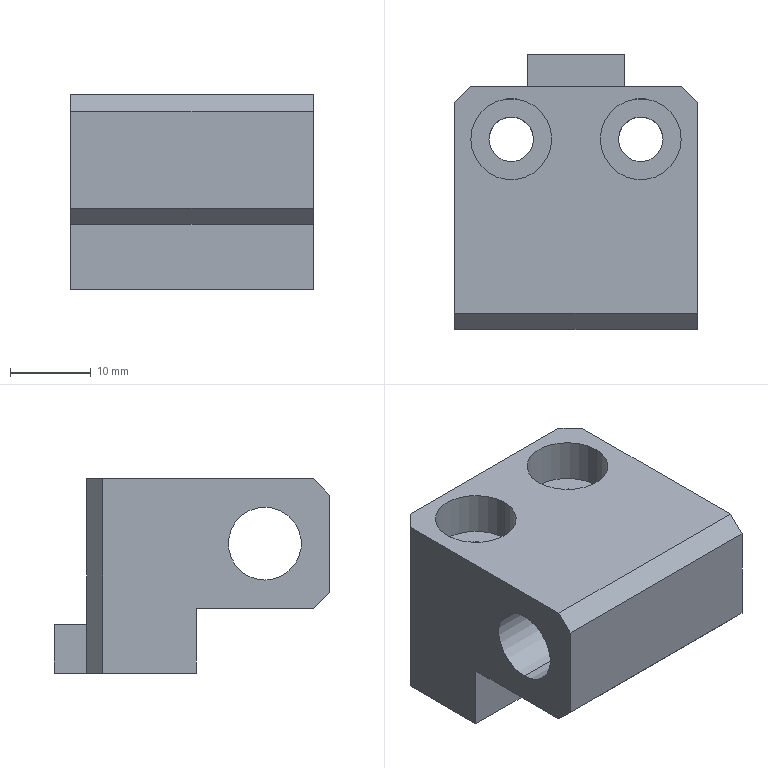Component | SolidWorks | 006GuideSeat-3 | 1 solid | 28 faces | box 30 x 34 x 24 mm | volume 14071 mm3 | plane 18 | cylinder 10 | commonest cylinder face diameters 10 x4 5.5 x4 9 x2
build123d program:
from build123d import *

# Parameters (mm, degrees)
SKETCH1_W                                            = 30
SKETCH1_H                                            = 30
BOSS_EXTRUDE1_DEPTH                                  = 24
SKETCH3_W                                            = 8
SKETCH3_H                                            = 16.5
CUT_EXTRUDE2_DEPTH                                   = 49.744
M5_HEX_SOCKET_HEAD_CAP_SCREW_COUNTERBORE_D           = 5.5
M5_HEX_SOCKET_HEAD_CAP_SCREW_COUNTERBORE_CBORE_D     = 10
M5_HEX_SOCKET_HEAD_CAP_SCREW_COUNTERBORE_CBORE_DEPTH = 5.4
SKETCH6_R                                            = 4.5
CUT_EXTRUDE3_DEPTH                                   = 49.744
CHAMFER1_SIZE                                        = 2
CHAMFER2_SIZE                                        = 2
SKETCH7_W                                            = 12
SKETCH7_H                                            = 6
BOSS_EXTRUDE2_DEPTH                                  = 4


with BuildPart() as part:
    # Sketch1 → Boss-Extrude1 (new body)
    with BuildSketch(Plane.XY):
        with Locations((15, 15)):
            Rectangle(SKETCH1_W, SKETCH1_H)
    extrude(amount=BOSS_EXTRUDE1_DEPTH)

    # Sketch3 → Cut-Extrude2 (cut, through all)
    with BuildSketch(Plane(origin=(30, 0, 0), x_dir=(0, 0, -1), z_dir=(1, 0, 0))):
        with Locations((-4, 8.25)):
            Rectangle(SKETCH3_W, SKETCH3_H)
    extrude(amount=-CUT_EXTRUDE2_DEPTH, mode=Mode.SUBTRACT)

    # M5 Hex Socket Head Cap Screw Counterbore (through all)
    with Locations(Plane.XY.offset(24)):
        with Locations((23, 23.5), (7, 23.5)):
            CounterBoreHole(M5_HEX_SOCKET_HEAD_CAP_SCREW_COUNTERBORE_D / 2, M5_HEX_SOCKET_HEAD_CAP_SCREW_COUNTERBORE_CBORE_D / 2, M5_HEX_SOCKET_HEAD_CAP_SCREW_COUNTERBORE_CBORE_DEPTH)

    # Sketch6 → Cut-Extrude3 (cut, through all)
    with BuildSketch(Plane(origin=(30, 0, 0), x_dir=(0, 0, -1), z_dir=(1, 0, 0))):
        with Locations((-16, 8)):
            Circle(SKETCH6_R)
    extrude(amount=-CUT_EXTRUDE3_DEPTH, mode=Mode.SUBTRACT)

    # Chamfer1
    chamfer1_edges = [part.edges().sort_by_distance(p)[0] for p in [
        (15, 0, 8),
        (15, 0, 24),
    ]]
    chamfer(chamfer1_edges, length=CHAMFER1_SIZE)

    # Chamfer2
    chamfer2_edges = [part.edges().sort_by_distance(p)[0] for p in [
        (0, 30, 12),
        (30, 30, 12),
    ]]
    chamfer(chamfer2_edges, length=CHAMFER2_SIZE)

    # Sketch7 → Boss-Extrude2 (add)
    with BuildSketch(Plane(origin=(0, 30, 0), x_dir=(1, 0, 0), z_dir=(0, 1, 0))):
        with Locations((15, -3)):
            Rectangle(SKETCH7_W, SKETCH7_H)
    extrude(amount=BOSS_EXTRUDE2_DEPTH)


solid = part.part

# Placed as in the assembly
solid = solid.moved(Location((-135.796, 16.924, 37.04), (0, 0, 0)))
STEP:
#1=CARTESIAN_POINT('',(-5.346,0.9813,2.265));
#2=VERTEX_POINT('',#1);
#3=CARTESIAN_POINT('',(-5.346,0.9813,1.911));
#4=VERTEX_POINT('',#3);
#5=CARTESIAN_POINT('',(-5.346,0.9813,2.088));
#6=DIRECTION('',(1.,0.,0.));
#7=DIRECTION('',(0.,0.,-1.));
#8=AXIS2_PLACEMENT_3D('',#5,#6,#7);
#9=CIRCLE('',#8,0.1772);
#10=EDGE_CURVE('',#2,#4,#9,.T.);
#11=ORIENTED_EDGE('',*,*,#10,.F.);
#12=CARTESIAN_POINT('',(-4.165,0.9813,2.265));
#13=VERTEX_POINT('',#12);
#14=CARTESIAN_POINT('',(-5.346,0.9813,2.265));
#15=DIRECTION('',(1.,0.,0.));
#16=VECTOR('',#15,39.37);
#17=LINE('',#14,#16);
#18=EDGE_CURVE('',#2,#13,#17,.T.);
#19=ORIENTED_EDGE('',*,*,#18,.T.);
#20=CARTESIAN_POINT('',(-4.165,0.9813,1.911));
#21=VERTEX_POINT('',#20);
#22=CARTESIAN_POINT('',(-4.165,0.9813,2.088));
#23=DIRECTION('',(1.,0.,0.));
#24=DIRECTION('',(0.,0.,-1.));
#25=AXIS2_PLACEMENT_3D('',#22,#23,#24);
#26=CIRCLE('',#25,0.1772);
#27=EDGE_CURVE('',#13,#21,#26,.T.);
#28=ORIENTED_EDGE('',*,*,#27,.T.);
#29=CARTESIAN_POINT('',(-5.346,0.9813,1.911));
#30=DIRECTION('',(1.,0.,0.));
#31=VECTOR('',#30,39.37);
#32=LINE('',#29,#31);
#33=EDGE_CURVE('',#4,#21,#32,.T.);
#34=ORIENTED_EDGE('',*,*,#33,.F.);
#35=EDGE_LOOP('',(#11,#19,#28,#34));
#36=FACE_OUTER_BOUND('',#35,.T.);
#37=CARTESIAN_POINT('',(-5.346,0.9813,2.088));
#38=DIRECTION('',(1.,0.,0.));
#39=DIRECTION('',(0.,0.,-1.));
#40=AXIS2_PLACEMENT_3D('',#37,#38,#39);
#41=CYLINDRICAL_SURFACE('',#40,0.1772);
#42=ADVANCED_FACE('',(#36),#41,.F.);
#43=CARTESIAN_POINT('',(-4.638,1.592,2.191));
#44=VERTEX_POINT('',#43);
#45=CARTESIAN_POINT('',(-4.244,1.592,2.191));
#46=VERTEX_POINT('',#45);
#47=CARTESIAN_POINT('',(-4.441,1.592,2.191));
#48=DIRECTION('',(0.,0.,1.));
#49=DIRECTION('',(1.,0.,0.));
#50=AXIS2_PLACEMENT_3D('',#47,#48,#49);
#51=CIRCLE('',#50,0.1969);
#52=EDGE_CURVE('',#44,#46,#51,.T.);
#53=ORIENTED_EDGE('',*,*,#52,.F.);
#54=CARTESIAN_POINT('',(-4.638,1.592,2.403));
#55=VERTEX_POINT('',#54);
#56=CARTESIAN_POINT('',(-4.638,1.592,2.403));
#57=DIRECTION('',(0.,0.,1.));
#58=VECTOR('',#57,39.37);
#59=LINE('',#56,#58);
#60=EDGE_CURVE('',#44,#55,#59,.T.);
#61=ORIENTED_EDGE('',*,*,#60,.T.);
#62=CARTESIAN_POINT('',(-4.244,1.592,2.403));
#63=VERTEX_POINT('',#62);
#64=CARTESIAN_POINT('',(-4.441,1.592,2.403));
#65=DIRECTION('',(0.,0.,1.));
#66=DIRECTION('',(1.,0.,0.));
#67=AXIS2_PLACEMENT_3D('',#64,#65,#66);
#68=CIRCLE('',#67,0.1969);
#69=EDGE_CURVE('',#55,#63,#68,.T.);
#70=ORIENTED_EDGE('',*,*,#69,.T.);
#71=CARTESIAN_POINT('',(-4.244,1.592,2.403));
#72=DIRECTION('',(0.,0.,1.));
#73=VECTOR('',#72,39.37);
#74=LINE('',#71,#73);
#75=EDGE_CURVE('',#46,#63,#74,.T.);
#76=ORIENTED_EDGE('',*,*,#75,.F.);
#77=EDGE_LOOP('',(#53,#61,#70,#76));
#78=FACE_OUTER_BOUND('',#77,.T.);
#79=CARTESIAN_POINT('',(-4.441,1.592,2.403));
#80=DIRECTION('',(0.,0.,1.));
#81=DIRECTION('',(1.,0.,0.));
#82=AXIS2_PLACEMENT_3D('',#79,#80,#81);
#83=CYLINDRICAL_SURFACE('',#82,0.1969);
#84=ADVANCED_FACE('',(#78),#83,.F.);
#85=CARTESIAN_POINT('',(-4.549,1.592,1.458));
#86=VERTEX_POINT('',#85);
#87=CARTESIAN_POINT('',(-4.333,1.592,1.458));
#88=VERTEX_POINT('',#87);
#89=CARTESIAN_POINT('',(-4.441,1.592,1.458));
#90=DIRECTION('',(0.,0.,1.));
#91=DIRECTION('',(1.,0.,0.));
#92=AXIS2_PLACEMENT_3D('',#89,#90,#91);
#93=CIRCLE('',#92,0.1083);
#94=EDGE_CURVE('',#86,#88,#93,.T.);
#95=ORIENTED_EDGE('',*,*,#94,.F.);
#96=CARTESIAN_POINT('',(-4.549,1.592,2.191));
#97=VERTEX_POINT('',#96);
#98=CARTESIAN_POINT('',(-4.549,1.592,2.403));
#99=DIRECTION('',(0.,0.,1.));
#100=VECTOR('',#99,39.37);
#101=LINE('',#98,#100);
#102=EDGE_CURVE('',#86,#97,#101,.T.);
#103=ORIENTED_EDGE('',*,*,#102,.T.);
#104=CARTESIAN_POINT('',(-4.333,1.592,2.191));
#105=VERTEX_POINT('',#104);
#106=CARTESIAN_POINT('',(-4.441,1.592,2.191));
#107=DIRECTION('',(0.,0.,1.));
#108=DIRECTION('',(1.,0.,0.));
#109=AXIS2_PLACEMENT_3D('',#106,#107,#108);
#110=CIRCLE('',#109,0.1083);
#111=EDGE_CURVE('',#97,#105,#110,.T.);
#112=ORIENTED_EDGE('',*,*,#111,.T.);
#113=CARTESIAN_POINT('',(-4.333,1.592,2.403));
#114=DIRECTION('',(0.,0.,1.));
#115=VECTOR('',#114,39.37);
#116=LINE('',#113,#115);
#117=EDGE_CURVE('',#88,#105,#116,.T.);
#118=ORIENTED_EDGE('',*,*,#117,.F.);
#119=EDGE_LOOP('',(#95,#103,#112,#118));
#120=FACE_OUTER_BOUND('',#119,.T.);
#121=CARTESIAN_POINT('',(-4.441,1.592,2.403));
#122=DIRECTION('',(0.,0.,1.));
#123=DIRECTION('',(1.,0.,0.));
#124=AXIS2_PLACEMENT_3D('',#121,#122,#123);
#125=CYLINDRICAL_SURFACE('',#124,0.1083);
#126=ADVANCED_FACE('',(#120),#125,.F.);
#127=CARTESIAN_POINT('',(-5.268,1.592,2.191));
#128=VERTEX_POINT('',#127);
#129=CARTESIAN_POINT('',(-4.874,1.592,2.191));
#130=VERTEX_POINT('',#129);
#131=CARTESIAN_POINT('',(-5.071,1.592,2.191));
#132=DIRECTION('',(0.,0.,1.));
#133=DIRECTION('',(1.,0.,0.));
#134=AXIS2_PLACEMENT_3D('',#131,#132,#133);
#135=CIRCLE('',#134,0.1969);
#136=EDGE_CURVE('',#128,#130,#135,.T.);
#137=ORIENTED_EDGE('',*,*,#136,.F.);
#138=CARTESIAN_POINT('',(-5.268,1.592,2.403));
#139=VERTEX_POINT('',#138);
#140=CARTESIAN_POINT('',(-5.268,1.592,2.403));
#141=DIRECTION('',(0.,0.,1.));
#142=VECTOR('',#141,39.37);
#143=LINE('',#140,#142);
#144=EDGE_CURVE('',#128,#139,#143,.T.);
#145=ORIENTED_EDGE('',*,*,#144,.T.);
#146=CARTESIAN_POINT('',(-4.874,1.592,2.403));
#147=VERTEX_POINT('',#146);
#148=CARTESIAN_POINT('',(-5.071,1.592,2.403));
#149=DIRECTION('',(0.,0.,1.));
#150=DIRECTION('',(1.,0.,0.));
#151=AXIS2_PLACEMENT_3D('',#148,#149,#150);
#152=CIRCLE('',#151,0.1969);
#153=EDGE_CURVE('',#139,#147,#152,.T.);
#154=ORIENTED_EDGE('',*,*,#153,.T.);
#155=CARTESIAN_POINT('',(-4.874,1.592,2.403));
#156=DIRECTION('',(0.,0.,1.));
#157=VECTOR('',#156,39.37);
#158=LINE('',#155,#157);
#159=EDGE_CURVE('',#130,#147,#158,.T.);
#160=ORIENTED_EDGE('',*,*,#159,.F.);
#161=EDGE_LOOP('',(#137,#145,#154,#160));
#162=FACE_OUTER_BOUND('',#161,.T.);
#163=CARTESIAN_POINT('',(-5.071,1.592,2.403));
#164=DIRECTION('',(0.,0.,1.));
#165=DIRECTION('',(1.,0.,0.));
#166=AXIS2_PLACEMENT_3D('',#163,#164,#165);
#167=CYLINDRICAL_SURFACE('',#166,0.1969);
#168=ADVANCED_FACE('',(#162),#167,.F.);
#169=CARTESIAN_POINT('',(-5.179,1.592,1.458));
#170=VERTEX_POINT('',#169);
#171=CARTESIAN_POINT('',(-4.962,1.592,1.458));
#172=VERTEX_POINT('',#171);
#173=CARTESIAN_POINT('',(-5.071,1.592,1.458));
#174=DIRECTION('',(0.,0.,1.));
#175=DIRECTION('',(1.,0.,0.));
#176=AXIS2_PLACEMENT_3D('',#173,#174,#175);
#177=CIRCLE('',#176,0.1083);
#178=EDGE_CURVE('',#170,#172,#177,.T.);
#179=ORIENTED_EDGE('',*,*,#178,.F.);
#180=CARTESIAN_POINT('',(-5.179,1.592,2.191));
#181=VERTEX_POINT('',#180);
#182=CARTESIAN_POINT('',(-5.179,1.592,2.403));
#183=DIRECTION('',(0.,0.,1.));
#184=VECTOR('',#183,39.37);
#185=LINE('',#182,#184);
#186=EDGE_CURVE('',#170,#181,#185,.T.);
#187=ORIENTED_EDGE('',*,*,#186,.T.);
#188=CARTESIAN_POINT('',(-4.962,1.592,2.191));
#189=VERTEX_POINT('',#188);
#190=CARTESIAN_POINT('',(-5.071,1.592,2.191));
#191=DIRECTION('',(0.,0.,1.));
#192=DIRECTION('',(1.,0.,0.));
#193=AXIS2_PLACEMENT_3D('',#190,#191,#192);
#194=CIRCLE('',#193,0.1083);
#195=EDGE_CURVE('',#181,#189,#194,.T.);
#196=ORIENTED_EDGE('',*,*,#195,.T.);
#197=CARTESIAN_POINT('',(-4.962,1.592,2.403));
#198=DIRECTION('',(0.,0.,1.));
#199=VECTOR('',#198,39.37);
#200=LINE('',#197,#199);
#201=EDGE_CURVE('',#172,#189,#200,.T.);
#202=ORIENTED_EDGE('',*,*,#201,.F.);
#203=EDGE_LOOP('',(#179,#187,#196,#202));
#204=FACE_OUTER_BOUND('',#203,.T.);
#205=CARTESIAN_POINT('',(-5.071,1.592,2.403));
#206=DIRECTION('',(0.,0.,1.));
#207=DIRECTION('',(1.,0.,0.));
#208=AXIS2_PLACEMENT_3D('',#205,#206,#207);
#209=CYLINDRICAL_SURFACE('',#208,0.1083);
#210=ADVANCED_FACE('',(#204),#209,.F.);
#211=CARTESIAN_POINT('',(-4.992,1.847,1.458));
#212=VERTEX_POINT('',#211);
#213=CARTESIAN_POINT('',(-4.992,1.847,1.695));
#214=VERTEX_POINT('',#213);
#215=CARTESIAN_POINT('',(-4.992,1.847,1.458));
#216=DIRECTION('',(0.,0.,1.));
#217=VECTOR('',#216,39.37);
#218=LINE('',#215,#217);
#219=EDGE_CURVE('',#212,#214,#218,.T.);
#220=ORIENTED_EDGE('',*,*,#219,.F.);
#221=CARTESIAN_POINT('',(-5.268,1.847,1.458));
#222=VERTEX_POINT('',#221);
#223=CARTESIAN_POINT('',(-5.346,1.847,1.458));
#224=DIRECTION('',(-1.,0.,0.));
#225=VECTOR('',#224,39.37);
#226=LINE('',#223,#225);
#227=EDGE_CURVE('',#212,#222,#226,.T.);
#228=ORIENTED_EDGE('',*,*,#227,.T.);
#229=CARTESIAN_POINT('',(-5.268,1.847,2.403));
#230=VERTEX_POINT('',#229);
#231=CARTESIAN_POINT('',(-5.268,1.847,2.403));
#232=DIRECTION('',(0.,0.,1.));
#233=VECTOR('',#232,39.37);
#234=LINE('',#231,#233);
#235=EDGE_CURVE('',#222,#230,#234,.T.);
#236=ORIENTED_EDGE('',*,*,#235,.T.);
#237=CARTESIAN_POINT('',(-4.244,1.847,2.403));
#238=VERTEX_POINT('',#237);
#239=CARTESIAN_POINT('',(-5.346,1.847,2.403));
#240=DIRECTION('',(-1.,0.,0.));
#241=VECTOR('',#240,39.37);
#242=LINE('',#239,#241);
#243=EDGE_CURVE('',#238,#230,#242,.T.);
#244=ORIENTED_EDGE('',*,*,#243,.F.);
#245=CARTESIAN_POINT('',(-4.244,1.847,1.458));
#246=VERTEX_POINT('',#245);
#247=CARTESIAN_POINT('',(-4.244,1.847,2.403));
#248=DIRECTION('',(0.,0.,-1.));
#249=VECTOR('',#248,39.37);
#250=LINE('',#247,#249);
#251=EDGE_CURVE('',#238,#246,#250,.T.);
#252=ORIENTED_EDGE('',*,*,#251,.T.);
#253=CARTESIAN_POINT('',(-4.52,1.847,1.458));
#254=VERTEX_POINT('',#253);
#255=CARTESIAN_POINT('',(-5.346,1.847,1.458));
#256=DIRECTION('',(-1.,0.,0.));
#257=VECTOR('',#256,39.37);
#258=LINE('',#255,#257);
#259=EDGE_CURVE('',#246,#254,#258,.T.);
#260=ORIENTED_EDGE('',*,*,#259,.T.);
#261=CARTESIAN_POINT('',(-4.52,1.847,1.695));
#262=VERTEX_POINT('',#261);
#263=CARTESIAN_POINT('',(-4.52,1.847,1.458));
#264=DIRECTION('',(0.,0.,-1.));
#265=VECTOR('',#264,39.37);
#266=LINE('',#263,#265);
#267=EDGE_CURVE('',#262,#254,#266,.T.);
#268=ORIENTED_EDGE('',*,*,#267,.F.);
#269=CARTESIAN_POINT('',(-4.992,1.847,1.695));
#270=DIRECTION('',(1.,0.,0.));
#271=VECTOR('',#270,39.37);
#272=LINE('',#269,#271);
#273=EDGE_CURVE('',#214,#262,#272,.T.);
#274=ORIENTED_EDGE('',*,*,#273,.F.);
#275=EDGE_LOOP('',(#220,#228,#236,#244,#252,#260,#268,#274));
#276=FACE_OUTER_BOUND('',#275,.T.);
#277=CARTESIAN_POINT('',(-5.346,1.847,2.403));
#278=DIRECTION('',(0.,-1.,0.));
#279=DIRECTION('',(0.,0.,-1.));
#280=AXIS2_PLACEMENT_3D('',#277,#278,#279);
#281=PLANE('',#280);
#282=ADVANCED_FACE('',(#276),#281,.F.);
#283=CARTESIAN_POINT('',(-5.346,0.9813,2.088));
#284=DIRECTION('',(1.,0.,0.));
#285=DIRECTION('',(0.,0.,-1.));
#286=AXIS2_PLACEMENT_3D('',#283,#284,#285);
#287=CIRCLE('',#286,0.1772);
#288=EDGE_CURVE('',#4,#2,#287,.T.);
#289=ORIENTED_EDGE('',*,*,#288,.T.);
#290=ORIENTED_EDGE('',*,*,#10,.T.);
#291=EDGE_LOOP('',(#289,#290));
#292=FACE_BOUND('',#291,.T.);
#293=CARTESIAN_POINT('',(-5.346,1.769,2.403));
#294=VERTEX_POINT('',#293);
#295=CARTESIAN_POINT('',(-5.346,0.7451,2.403));
#296=VERTEX_POINT('',#295);
#297=CARTESIAN_POINT('',(-5.346,0.6663,2.403));
#298=DIRECTION('',(0.,-1.,0.));
#299=VECTOR('',#298,39.37);
#300=LINE('',#297,#299);
#301=EDGE_CURVE('',#294,#296,#300,.T.);
#302=ORIENTED_EDGE('',*,*,#301,.F.);
#303=CARTESIAN_POINT('',(-5.346,1.769,1.458));
#304=VERTEX_POINT('',#303);
#305=CARTESIAN_POINT('',(-5.346,1.769,2.403));
#306=DIRECTION('',(0.,0.,-1.));
#307=VECTOR('',#306,39.37);
#308=LINE('',#305,#307);
#309=EDGE_CURVE('',#294,#304,#308,.T.);
#310=ORIENTED_EDGE('',*,*,#309,.T.);
#311=CARTESIAN_POINT('',(-5.346,1.316,1.458));
#312=VERTEX_POINT('',#311);
#313=CARTESIAN_POINT('',(-5.346,0.6663,1.458));
#314=DIRECTION('',(0.,-1.,0.));
#315=VECTOR('',#314,39.37);
#316=LINE('',#313,#315);
#317=EDGE_CURVE('',#304,#312,#316,.T.);
#318=ORIENTED_EDGE('',*,*,#317,.T.);
#319=CARTESIAN_POINT('',(-5.346,1.316,1.773));
#320=VERTEX_POINT('',#319);
#321=CARTESIAN_POINT('',(-5.346,1.316,1.458));
#322=DIRECTION('',(0.,0.,1.));
#323=VECTOR('',#322,39.37);
#324=LINE('',#321,#323);
#325=EDGE_CURVE('',#312,#320,#324,.T.);
#326=ORIENTED_EDGE('',*,*,#325,.T.);
#327=CARTESIAN_POINT('',(-5.346,0.7451,1.773));
#328=VERTEX_POINT('',#327);
#329=CARTESIAN_POINT('',(-5.346,0.6663,1.773));
#330=DIRECTION('',(0.,-1.,0.));
#331=VECTOR('',#330,39.37);
#332=LINE('',#329,#331);
#333=EDGE_CURVE('',#320,#328,#332,.T.);
#334=ORIENTED_EDGE('',*,*,#333,.T.);
#335=CARTESIAN_POINT('',(-5.346,0.6663,1.852));
#336=VERTEX_POINT('',#335);
#337=CARTESIAN_POINT('',(-5.346,0.6663,1.852));
#338=DIRECTION('',(0.,-0.7071,0.7071));
#339=VECTOR('',#338,39.37);
#340=LINE('',#337,#339);
#341=EDGE_CURVE('',#328,#336,#340,.T.);
#342=ORIENTED_EDGE('',*,*,#341,.T.);
#343=CARTESIAN_POINT('',(-5.346,0.6663,2.324));
#344=VERTEX_POINT('',#343);
#345=CARTESIAN_POINT('',(-5.346,0.6663,2.403));
#346=DIRECTION('',(0.,0.,-1.));
#347=VECTOR('',#346,39.37);
#348=LINE('',#345,#347);
#349=EDGE_CURVE('',#344,#336,#348,.T.);
#350=ORIENTED_EDGE('',*,*,#349,.F.);
#351=CARTESIAN_POINT('',(-5.346,0.7451,2.403));
#352=DIRECTION('',(0.,0.7071,0.7071));
#353=VECTOR('',#352,39.37);
#354=LINE('',#351,#353);
#355=EDGE_CURVE('',#344,#296,#354,.T.);
#356=ORIENTED_EDGE('',*,*,#355,.T.);
#357=EDGE_LOOP('',(#302,#310,#318,#326,#334,#342,#350,#356));
#358=FACE_OUTER_BOUND('',#357,.T.);
#359=CARTESIAN_POINT('',(-5.346,0.6663,2.403));
#360=DIRECTION('',(1.,0.,0.));
#361=DIRECTION('',(0.,0.,-1.));
#362=AXIS2_PLACEMENT_3D('',#359,#360,#361);
#363=PLANE('',#362);
#364=ADVANCED_FACE('',(#292,#358),#363,.F.);
#365=ORIENTED_EDGE('',*,*,#349,.T.);
#366=CARTESIAN_POINT('',(-4.165,0.6663,1.852));
#367=VERTEX_POINT('',#366);
#368=CARTESIAN_POINT('',(-5.346,0.6663,1.852));
#369=DIRECTION('',(1.,0.,0.));
#370=VECTOR('',#369,39.37);
#371=LINE('',#368,#370);
#372=EDGE_CURVE('',#336,#367,#371,.T.);
#373=ORIENTED_EDGE('',*,*,#372,.T.);
#374=CARTESIAN_POINT('',(-4.165,0.6663,2.324));
#375=VERTEX_POINT('',#374);
#376=CARTESIAN_POINT('',(-4.165,0.6663,2.403));
#377=DIRECTION('',(0.,0.,-1.));
#378=VECTOR('',#377,39.37);
#379=LINE('',#376,#378);
#380=EDGE_CURVE('',#375,#367,#379,.T.);
#381=ORIENTED_EDGE('',*,*,#380,.F.);
#382=CARTESIAN_POINT('',(-5.346,0.6663,2.324));
#383=DIRECTION('',(-1.,0.,0.));
#384=VECTOR('',#383,39.37);
#385=LINE('',#382,#384);
#386=EDGE_CURVE('',#375,#344,#385,.T.);
#387=ORIENTED_EDGE('',*,*,#386,.T.);
#388=EDGE_LOOP('',(#365,#373,#381,#387));
#389=FACE_OUTER_BOUND('',#388,.T.);
#390=CARTESIAN_POINT('',(-5.346,0.6663,2.403));
#391=DIRECTION('',(0.,1.,0.));
#392=DIRECTION('',(0.,0.,1.));
#393=AXIS2_PLACEMENT_3D('',#390,#391,#392);
#394=PLANE('',#393);
#395=ADVANCED_FACE('',(#389),#394,.F.);
#396=CARTESIAN_POINT('',(-4.165,0.9813,2.088));
#397=DIRECTION('',(1.,0.,0.));
#398=DIRECTION('',(0.,0.,-1.));
#399=AXIS2_PLACEMENT_3D('',#396,#397,#398);
#400=CIRCLE('',#399,0.1772);
#401=EDGE_CURVE('',#21,#13,#400,.T.);
#402=ORIENTED_EDGE('',*,*,#401,.F.);
#403=ORIENTED_EDGE('',*,*,#27,.F.);
#404=EDGE_LOOP('',(#402,#403));
#405=FACE_BOUND('',#404,.T.);
#406=CARTESIAN_POINT('',(-4.165,1.316,1.458));
#407=VERTEX_POINT('',#406);
#408=CARTESIAN_POINT('',(-4.165,1.769,1.458));
#409=VERTEX_POINT('',#408);
#410=CARTESIAN_POINT('',(-4.165,0.6663,1.458));
#411=DIRECTION('',(0.,1.,0.));
#412=VECTOR('',#411,39.37);
#413=LINE('',#410,#412);
#414=EDGE_CURVE('',#407,#409,#413,.T.);
#415=ORIENTED_EDGE('',*,*,#414,.T.);
#416=CARTESIAN_POINT('',(-4.165,1.769,2.403));
#417=VERTEX_POINT('',#416);
#418=CARTESIAN_POINT('',(-4.165,1.769,2.403));
#419=DIRECTION('',(0.,0.,1.));
#420=VECTOR('',#419,39.37);
#421=LINE('',#418,#420);
#422=EDGE_CURVE('',#409,#417,#421,.T.);
#423=ORIENTED_EDGE('',*,*,#422,.T.);
#424=CARTESIAN_POINT('',(-4.165,0.7451,2.403));
#425=VERTEX_POINT('',#424);
#426=CARTESIAN_POINT('',(-4.165,0.6663,2.403));
#427=DIRECTION('',(0.,1.,0.));
#428=VECTOR('',#427,39.37);
#429=LINE('',#426,#428);
#430=EDGE_CURVE('',#425,#417,#429,.T.);
#431=ORIENTED_EDGE('',*,*,#430,.F.);
#432=CARTESIAN_POINT('',(-4.165,0.7451,2.403));
#433=DIRECTION('',(0.,-0.7071,-0.7071));
#434=VECTOR('',#433,39.37);
#435=LINE('',#432,#434);
#436=EDGE_CURVE('',#425,#375,#435,.T.);
#437=ORIENTED_EDGE('',*,*,#436,.T.);
#438=ORIENTED_EDGE('',*,*,#380,.T.);
#439=CARTESIAN_POINT('',(-4.165,0.7451,1.773));
#440=VERTEX_POINT('',#439);
#441=CARTESIAN_POINT('',(-4.165,0.6663,1.852));
#442=DIRECTION('',(0.,0.7071,-0.7071));
#443=VECTOR('',#442,39.37);
#444=LINE('',#441,#443);
#445=EDGE_CURVE('',#367,#440,#444,.T.);
#446=ORIENTED_EDGE('',*,*,#445,.T.);
#447=CARTESIAN_POINT('',(-4.165,1.316,1.773));
#448=VERTEX_POINT('',#447);
#449=CARTESIAN_POINT('',(-4.165,0.6663,1.773));
#450=DIRECTION('',(0.,-1.,0.));
#451=VECTOR('',#450,39.37);
#452=LINE('',#449,#451);
#453=EDGE_CURVE('',#448,#440,#452,.T.);
#454=ORIENTED_EDGE('',*,*,#453,.F.);
#455=CARTESIAN_POINT('',(-4.165,1.316,1.458));
#456=DIRECTION('',(0.,0.,1.));
#457=VECTOR('',#456,39.37);
#458=LINE('',#455,#457);
#459=EDGE_CURVE('',#407,#448,#458,.T.);
#460=ORIENTED_EDGE('',*,*,#459,.F.);
#461=EDGE_LOOP('',(#415,#423,#431,#437,#438,#446,#454,#460));
#462=FACE_OUTER_BOUND('',#461,.T.);
#463=CARTESIAN_POINT('',(-4.165,0.6663,2.403));
#464=DIRECTION('',(-1.,0.,0.));
#465=DIRECTION('',(0.,0.,1.));
#466=AXIS2_PLACEMENT_3D('',#463,#464,#465);
#467=PLANE('',#466);
#468=ADVANCED_FACE('',(#405,#462),#467,.F.);
#469=CARTESIAN_POINT('',(-4.441,1.592,2.403));
#470=DIRECTION('',(0.,0.,1.));
#471=DIRECTION('',(1.,0.,0.));
#472=AXIS2_PLACEMENT_3D('',#469,#470,#471);
#473=CIRCLE('',#472,0.1969);
#474=EDGE_CURVE('',#63,#55,#473,.T.);
#475=ORIENTED_EDGE('',*,*,#474,.F.);
#476=ORIENTED_EDGE('',*,*,#69,.F.);
#477=EDGE_LOOP('',(#475,#476));
#478=FACE_BOUND('',#477,.T.);
#479=CARTESIAN_POINT('',(-5.071,1.592,2.403));
#480=DIRECTION('',(0.,0.,1.));
#481=DIRECTION('',(1.,0.,0.));
#482=AXIS2_PLACEMENT_3D('',#479,#480,#481);
#483=CIRCLE('',#482,0.1969);
#484=EDGE_CURVE('',#147,#139,#483,.T.);
#485=ORIENTED_EDGE('',*,*,#484,.F.);
#486=ORIENTED_EDGE('',*,*,#153,.F.);
#487=EDGE_LOOP('',(#485,#486));
#488=FACE_BOUND('',#487,.T.);
#489=ORIENTED_EDGE('',*,*,#243,.T.);
#490=CARTESIAN_POINT('',(-5.346,1.769,2.403));
#491=DIRECTION('',(-0.7071,-0.7071,0.));
#492=VECTOR('',#491,39.37);
#493=LINE('',#490,#492);
#494=EDGE_CURVE('',#230,#294,#493,.T.);
#495=ORIENTED_EDGE('',*,*,#494,.T.);
#496=ORIENTED_EDGE('',*,*,#301,.T.);
#497=CARTESIAN_POINT('',(-5.346,0.7451,2.403));
#498=DIRECTION('',(1.,0.,0.));
#499=VECTOR('',#498,39.37);
#500=LINE('',#497,#499);
#501=EDGE_CURVE('',#296,#425,#500,.T.);
#502=ORIENTED_EDGE('',*,*,#501,.T.);
#503=ORIENTED_EDGE('',*,*,#430,.T.);
#504=CARTESIAN_POINT('',(-4.244,1.847,2.403));
#505=DIRECTION('',(-0.7071,0.7071,0.));
#506=VECTOR('',#505,39.37);
#507=LINE('',#504,#506);
#508=EDGE_CURVE('',#417,#238,#507,.T.);
#509=ORIENTED_EDGE('',*,*,#508,.T.);
#510=EDGE_LOOP('',(#489,#495,#496,#502,#503,#509));
#511=FACE_OUTER_BOUND('',#510,.T.);
#512=CARTESIAN_POINT('',(-5.346,0.6663,2.403));
#513=DIRECTION('',(0.,0.,-1.));
#514=DIRECTION('',(-1.,0.,0.));
#515=AXIS2_PLACEMENT_3D('',#512,#513,#514);
#516=PLANE('',#515);
#517=ADVANCED_FACE('',(#478,#488,#511),#516,.F.);
#518=CARTESIAN_POINT('',(-4.441,1.592,1.458));
#519=DIRECTION('',(0.,0.,1.));
#520=DIRECTION('',(1.,0.,0.));
#521=AXIS2_PLACEMENT_3D('',#518,#519,#520);
#522=CIRCLE('',#521,0.1083);
#523=EDGE_CURVE('',#88,#86,#522,.T.);
#524=ORIENTED_EDGE('',*,*,#523,.T.);
#525=ORIENTED_EDGE('',*,*,#94,.T.);
#526=EDGE_LOOP('',(#524,#525));
#527=FACE_BOUND('',#526,.T.);
#528=CARTESIAN_POINT('',(-5.071,1.592,1.458));
#529=DIRECTION('',(0.,0.,1.));
#530=DIRECTION('',(1.,0.,0.));
#531=AXIS2_PLACEMENT_3D('',#528,#529,#530);
#532=CIRCLE('',#531,0.1083);
#533=EDGE_CURVE('',#172,#170,#532,.T.);
#534=ORIENTED_EDGE('',*,*,#533,.T.);
#535=ORIENTED_EDGE('',*,*,#178,.T.);
#536=EDGE_LOOP('',(#534,#535));
#537=FACE_BOUND('',#536,.T.);
#538=ORIENTED_EDGE('',*,*,#317,.F.);
#539=CARTESIAN_POINT('',(-5.897,1.217,1.458));
#540=DIRECTION('',(0.7071,0.7071,0.));
#541=VECTOR('',#540,39.37);
#542=LINE('',#539,#541);
#543=EDGE_CURVE('',#304,#222,#542,.T.);
#544=ORIENTED_EDGE('',*,*,#543,.T.);
#545=ORIENTED_EDGE('',*,*,#227,.F.);
#546=CARTESIAN_POINT('',(-4.992,2.005,1.458));
#547=VERTEX_POINT('',#546);
#548=CARTESIAN_POINT('',(-4.992,2.005,1.458));
#549=DIRECTION('',(0.,-1.,0.));
#550=VECTOR('',#549,39.37);
#551=LINE('',#548,#550);
#552=EDGE_CURVE('',#547,#212,#551,.T.);
#553=ORIENTED_EDGE('',*,*,#552,.F.);
#554=CARTESIAN_POINT('',(-4.52,2.005,1.458));
#555=VERTEX_POINT('',#554);
#556=CARTESIAN_POINT('',(-4.992,2.005,1.458));
#557=DIRECTION('',(-1.,0.,0.));
#558=VECTOR('',#557,39.37);
#559=LINE('',#556,#558);
#560=EDGE_CURVE('',#555,#547,#559,.T.);
#561=ORIENTED_EDGE('',*,*,#560,.F.);
#562=CARTESIAN_POINT('',(-4.52,2.005,1.458));
#563=DIRECTION('',(0.,-1.,0.));
#564=VECTOR('',#563,39.37);
#565=LINE('',#562,#564);
#566=EDGE_CURVE('',#555,#254,#565,.T.);
#567=ORIENTED_EDGE('',*,*,#566,.T.);
#568=ORIENTED_EDGE('',*,*,#259,.F.);
#569=CARTESIAN_POINT('',(-4.205,1.808,1.458));
#570=DIRECTION('',(0.7071,-0.7071,0.));
#571=VECTOR('',#570,39.37);
#572=LINE('',#569,#571);
#573=EDGE_CURVE('',#246,#409,#572,.T.);
#574=ORIENTED_EDGE('',*,*,#573,.T.);
#575=ORIENTED_EDGE('',*,*,#414,.F.);
#576=CARTESIAN_POINT('',(-5.346,1.316,1.458));
#577=DIRECTION('',(1.,0.,0.));
#578=VECTOR('',#577,39.37);
#579=LINE('',#576,#578);
#580=EDGE_CURVE('',#312,#407,#579,.T.);
#581=ORIENTED_EDGE('',*,*,#580,.F.);
#582=EDGE_LOOP('',(#538,#544,#545,#553,#561,#567,#568,#574,#575,#581));
#583=FACE_OUTER_BOUND('',#582,.T.);
#584=CARTESIAN_POINT('',(-5.346,0.6663,1.458));
#585=DIRECTION('',(0.,0.,-1.));
#586=DIRECTION('',(-1.,0.,0.));
#587=AXIS2_PLACEMENT_3D('',#584,#585,#586);
#588=PLANE('',#587);
#589=ADVANCED_FACE('',(#527,#537,#583),#588,.T.);
#590=ORIENTED_EDGE('',*,*,#453,.T.);
#591=CARTESIAN_POINT('',(-5.346,0.7451,1.773));
#592=DIRECTION('',(-1.,0.,0.));
#593=VECTOR('',#592,39.37);
#594=LINE('',#591,#593);
#595=EDGE_CURVE('',#440,#328,#594,.T.);
#596=ORIENTED_EDGE('',*,*,#595,.T.);
#597=ORIENTED_EDGE('',*,*,#333,.F.);
#598=CARTESIAN_POINT('',(-5.346,1.316,1.773));
#599=DIRECTION('',(1.,0.,0.));
#600=VECTOR('',#599,39.37);
#601=LINE('',#598,#600);
#602=EDGE_CURVE('',#320,#448,#601,.T.);
#603=ORIENTED_EDGE('',*,*,#602,.T.);
#604=EDGE_LOOP('',(#590,#596,#597,#603));
#605=FACE_OUTER_BOUND('',#604,.T.);
#606=CARTESIAN_POINT('',(-5.346,0.6663,1.773));
#607=DIRECTION('',(0.,0.,1.));
#608=DIRECTION('',(1.,0.,0.));
#609=AXIS2_PLACEMENT_3D('',#606,#607,#608);
#610=PLANE('',#609);
#611=ADVANCED_FACE('',(#605),#610,.F.);
#612=ORIENTED_EDGE('',*,*,#459,.T.);
#613=ORIENTED_EDGE('',*,*,#602,.F.);
#614=ORIENTED_EDGE('',*,*,#325,.F.);
#615=ORIENTED_EDGE('',*,*,#580,.T.);
#616=EDGE_LOOP('',(#612,#613,#614,#615));
#617=FACE_OUTER_BOUND('',#616,.T.);
#618=CARTESIAN_POINT('',(-5.346,1.316,1.458));
#619=DIRECTION('',(0.,1.,0.));
#620=DIRECTION('',(0.,0.,1.));
#621=AXIS2_PLACEMENT_3D('',#618,#619,#620);
#622=PLANE('',#621);
#623=ADVANCED_FACE('',(#617),#622,.F.);
#624=ORIENTED_EDGE('',*,*,#186,.F.);
#625=ORIENTED_EDGE('',*,*,#533,.F.);
#626=ORIENTED_EDGE('',*,*,#201,.T.);
#627=CARTESIAN_POINT('',(-5.071,1.592,2.191));
#628=DIRECTION('',(0.,0.,1.));
#629=DIRECTION('',(1.,0.,0.));
#630=AXIS2_PLACEMENT_3D('',#627,#628,#629);
#631=CIRCLE('',#630,0.1083);
#632=EDGE_CURVE('',#189,#181,#631,.T.);
#633=ORIENTED_EDGE('',*,*,#632,.T.);
#634=EDGE_LOOP('',(#624,#625,#626,#633));
#635=FACE_OUTER_BOUND('',#634,.T.);
#636=CARTESIAN_POINT('',(-5.071,1.592,2.403));
#637=DIRECTION('',(0.,0.,1.));
#638=DIRECTION('',(1.,0.,0.));
#639=AXIS2_PLACEMENT_3D('',#636,#637,#638);
#640=CYLINDRICAL_SURFACE('',#639,0.1083);
#641=ADVANCED_FACE('',(#635),#640,.F.);
#642=ORIENTED_EDGE('',*,*,#632,.F.);
#643=ORIENTED_EDGE('',*,*,#195,.F.);
#644=EDGE_LOOP('',(#642,#643));
#645=FACE_BOUND('',#644,.T.);
#646=CARTESIAN_POINT('',(-5.071,1.592,2.191));
#647=DIRECTION('',(0.,0.,1.));
#648=DIRECTION('',(1.,0.,0.));
#649=AXIS2_PLACEMENT_3D('',#646,#647,#648);
#650=CIRCLE('',#649,0.1969);
#651=EDGE_CURVE('',#130,#128,#650,.T.);
#652=ORIENTED_EDGE('',*,*,#651,.T.);
#653=ORIENTED_EDGE('',*,*,#136,.T.);
#654=EDGE_LOOP('',(#652,#653));
#655=FACE_OUTER_BOUND('',#654,.T.);
#656=CARTESIAN_POINT('',(-4.962,1.592,2.191));
#657=DIRECTION('',(0.,0.,-1.));
#658=DIRECTION('',(-1.,0.,0.));
#659=AXIS2_PLACEMENT_3D('',#656,#657,#658);
#660=PLANE('',#659);
#661=ADVANCED_FACE('',(#645,#655),#660,.F.);
#662=ORIENTED_EDGE('',*,*,#144,.F.);
#663=ORIENTED_EDGE('',*,*,#651,.F.);
#664=ORIENTED_EDGE('',*,*,#159,.T.);
#665=ORIENTED_EDGE('',*,*,#484,.T.);
#666=EDGE_LOOP('',(#662,#663,#664,#665));
#667=FACE_OUTER_BOUND('',#666,.T.);
#668=CARTESIAN_POINT('',(-5.071,1.592,2.403));
#669=DIRECTION('',(0.,0.,1.));
#670=DIRECTION('',(1.,0.,0.));
#671=AXIS2_PLACEMENT_3D('',#668,#669,#670);
#672=CYLINDRICAL_SURFACE('',#671,0.1969);
#673=ADVANCED_FACE('',(#667),#672,.F.);
#674=ORIENTED_EDGE('',*,*,#102,.F.);
#675=ORIENTED_EDGE('',*,*,#523,.F.);
#676=ORIENTED_EDGE('',*,*,#117,.T.);
#677=CARTESIAN_POINT('',(-4.441,1.592,2.191));
#678=DIRECTION('',(0.,0.,1.));
#679=DIRECTION('',(1.,0.,0.));
#680=AXIS2_PLACEMENT_3D('',#677,#678,#679);
#681=CIRCLE('',#680,0.1083);
#682=EDGE_CURVE('',#105,#97,#681,.T.);
#683=ORIENTED_EDGE('',*,*,#682,.T.);
#684=EDGE_LOOP('',(#674,#675,#676,#683));
#685=FACE_OUTER_BOUND('',#684,.T.);
#686=CARTESIAN_POINT('',(-4.441,1.592,2.403));
#687=DIRECTION('',(0.,0.,1.));
#688=DIRECTION('',(1.,0.,0.));
#689=AXIS2_PLACEMENT_3D('',#686,#687,#688);
#690=CYLINDRICAL_SURFACE('',#689,0.1083);
#691=ADVANCED_FACE('',(#685),#690,.F.);
#692=ORIENTED_EDGE('',*,*,#682,.F.);
#693=ORIENTED_EDGE('',*,*,#111,.F.);
#694=EDGE_LOOP('',(#692,#693));
#695=FACE_BOUND('',#694,.T.);
#696=CARTESIAN_POINT('',(-4.441,1.592,2.191));
#697=DIRECTION('',(0.,0.,1.));
#698=DIRECTION('',(1.,0.,0.));
#699=AXIS2_PLACEMENT_3D('',#696,#697,#698);
#700=CIRCLE('',#699,0.1969);
#701=EDGE_CURVE('',#46,#44,#700,.T.);
#702=ORIENTED_EDGE('',*,*,#701,.T.);
#703=ORIENTED_EDGE('',*,*,#52,.T.);
#704=EDGE_LOOP('',(#702,#703));
#705=FACE_OUTER_BOUND('',#704,.T.);
#706=CARTESIAN_POINT('',(-4.333,1.592,2.191));
#707=DIRECTION('',(0.,0.,-1.));
#708=DIRECTION('',(-1.,0.,0.));
#709=AXIS2_PLACEMENT_3D('',#706,#707,#708);
#710=PLANE('',#709);
#711=ADVANCED_FACE('',(#695,#705),#710,.F.);
#712=ORIENTED_EDGE('',*,*,#60,.F.);
#713=ORIENTED_EDGE('',*,*,#701,.F.);
#714=ORIENTED_EDGE('',*,*,#75,.T.);
#715=ORIENTED_EDGE('',*,*,#474,.T.);
#716=EDGE_LOOP('',(#712,#713,#714,#715));
#717=FACE_OUTER_BOUND('',#716,.T.);
#718=CARTESIAN_POINT('',(-4.441,1.592,2.403));
#719=DIRECTION('',(0.,0.,1.));
#720=DIRECTION('',(1.,0.,0.));
#721=AXIS2_PLACEMENT_3D('',#718,#719,#720);
#722=CYLINDRICAL_SURFACE('',#721,0.1969);
#723=ADVANCED_FACE('',(#717),#722,.F.);
#724=ORIENTED_EDGE('',*,*,#18,.F.);
#725=ORIENTED_EDGE('',*,*,#288,.F.);
#726=ORIENTED_EDGE('',*,*,#33,.T.);
#727=ORIENTED_EDGE('',*,*,#401,.T.);
#728=EDGE_LOOP('',(#724,#725,#726,#727));
#729=FACE_OUTER_BOUND('',#728,.T.);
#730=CARTESIAN_POINT('',(-5.346,0.9813,2.088));
#731=DIRECTION('',(1.,0.,0.));
#732=DIRECTION('',(0.,0.,-1.));
#733=AXIS2_PLACEMENT_3D('',#730,#731,#732);
#734=CYLINDRICAL_SURFACE('',#733,0.1772);
#735=ADVANCED_FACE('',(#729),#734,.F.);
#736=ORIENTED_EDGE('',*,*,#341,.F.);
#737=ORIENTED_EDGE('',*,*,#595,.F.);
#738=ORIENTED_EDGE('',*,*,#445,.F.);
#739=ORIENTED_EDGE('',*,*,#372,.F.);
#740=EDGE_LOOP('',(#736,#737,#738,#739));
#741=FACE_OUTER_BOUND('',#740,.T.);
#742=CARTESIAN_POINT('',(-5.346,0.6663,1.852));
#743=DIRECTION('',(0.,0.7071,0.7071));
#744=DIRECTION('',(1.,0.,0.));
#745=AXIS2_PLACEMENT_3D('',#742,#743,#744);
#746=PLANE('',#745);
#747=ADVANCED_FACE('',(#741),#746,.F.);
#748=ORIENTED_EDGE('',*,*,#355,.F.);
#749=ORIENTED_EDGE('',*,*,#386,.F.);
#750=ORIENTED_EDGE('',*,*,#436,.F.);
#751=ORIENTED_EDGE('',*,*,#501,.F.);
#752=EDGE_LOOP('',(#748,#749,#750,#751));
#753=FACE_OUTER_BOUND('',#752,.T.);
#754=CARTESIAN_POINT('',(-5.346,0.7451,2.403));
#755=DIRECTION('',(0.,0.7071,-0.7071));
#756=DIRECTION('',(1.,0.,0.));
#757=AXIS2_PLACEMENT_3D('',#754,#755,#756);
#758=PLANE('',#757);
#759=ADVANCED_FACE('',(#753),#758,.F.);
#760=ORIENTED_EDGE('',*,*,#494,.F.);
#761=ORIENTED_EDGE('',*,*,#235,.F.);
#762=ORIENTED_EDGE('',*,*,#543,.F.);
#763=ORIENTED_EDGE('',*,*,#309,.F.);
#764=EDGE_LOOP('',(#760,#761,#762,#763));
#765=FACE_OUTER_BOUND('',#764,.T.);
#766=CARTESIAN_POINT('',(-5.346,1.769,2.403));
#767=DIRECTION('',(0.7071,-0.7071,0.));
#768=DIRECTION('',(0.,0.,-1.));
#769=AXIS2_PLACEMENT_3D('',#766,#767,#768);
#770=PLANE('',#769);
#771=ADVANCED_FACE('',(#765),#770,.F.);
#772=ORIENTED_EDGE('',*,*,#508,.F.);
#773=ORIENTED_EDGE('',*,*,#422,.F.);
#774=ORIENTED_EDGE('',*,*,#573,.F.);
#775=ORIENTED_EDGE('',*,*,#251,.F.);
#776=EDGE_LOOP('',(#772,#773,#774,#775));
#777=FACE_OUTER_BOUND('',#776,.T.);
#778=CARTESIAN_POINT('',(-4.244,1.847,2.403));
#779=DIRECTION('',(-0.7071,-0.7071,0.));
#780=DIRECTION('',(0.,0.,-1.));
#781=AXIS2_PLACEMENT_3D('',#778,#779,#780);
#782=PLANE('',#781);
#783=ADVANCED_FACE('',(#777),#782,.F.);
#784=ORIENTED_EDGE('',*,*,#219,.T.);
#785=CARTESIAN_POINT('',(-4.992,2.005,1.695));
#786=VERTEX_POINT('',#785);
#787=CARTESIAN_POINT('',(-4.992,2.005,1.695));
#788=DIRECTION('',(0.,-1.,0.));
#789=VECTOR('',#788,39.37);
#790=LINE('',#787,#789);
#791=EDGE_CURVE('',#786,#214,#790,.T.);
#792=ORIENTED_EDGE('',*,*,#791,.F.);
#793=CARTESIAN_POINT('',(-4.992,2.005,1.458));
#794=DIRECTION('',(0.,0.,1.));
#795=VECTOR('',#794,39.37);
#796=LINE('',#793,#795);
#797=EDGE_CURVE('',#547,#786,#796,.T.);
#798=ORIENTED_EDGE('',*,*,#797,.F.);
#799=ORIENTED_EDGE('',*,*,#552,.T.);
#800=EDGE_LOOP('',(#784,#792,#798,#799));
#801=FACE_OUTER_BOUND('',#800,.T.);
#802=CARTESIAN_POINT('',(-4.992,2.005,1.458));
#803=DIRECTION('',(1.,0.,-0.));
#804=DIRECTION('',(-0.,0.,-1.));
#805=AXIS2_PLACEMENT_3D('',#802,#803,#804);
#806=PLANE('',#805);
#807=ADVANCED_FACE('',(#801),#806,.F.);
#808=ORIENTED_EDGE('',*,*,#273,.T.);
#809=CARTESIAN_POINT('',(-4.52,2.005,1.695));
#810=VERTEX_POINT('',#809);
#811=CARTESIAN_POINT('',(-4.52,2.005,1.695));
#812=DIRECTION('',(0.,-1.,0.));
#813=VECTOR('',#812,39.37);
#814=LINE('',#811,#813);
#815=EDGE_CURVE('',#810,#262,#814,.T.);
#816=ORIENTED_EDGE('',*,*,#815,.F.);
#817=CARTESIAN_POINT('',(-4.992,2.005,1.695));
#818=DIRECTION('',(1.,0.,0.));
#819=VECTOR('',#818,39.37);
#820=LINE('',#817,#819);
#821=EDGE_CURVE('',#786,#810,#820,.T.);
#822=ORIENTED_EDGE('',*,*,#821,.F.);
#823=ORIENTED_EDGE('',*,*,#791,.T.);
#824=EDGE_LOOP('',(#808,#816,#822,#823));
#825=FACE_OUTER_BOUND('',#824,.T.);
#826=CARTESIAN_POINT('',(-4.992,2.005,1.695));
#827=DIRECTION('',(0.,0.,-1.));
#828=DIRECTION('',(-1.,0.,0.));
#829=AXIS2_PLACEMENT_3D('',#826,#827,#828);
#830=PLANE('',#829);
#831=ADVANCED_FACE('',(#825),#830,.F.);
#832=ORIENTED_EDGE('',*,*,#267,.T.);
#833=ORIENTED_EDGE('',*,*,#566,.F.);
#834=CARTESIAN_POINT('',(-4.52,2.005,1.458));
#835=DIRECTION('',(0.,0.,-1.));
#836=VECTOR('',#835,39.37);
#837=LINE('',#834,#836);
#838=EDGE_CURVE('',#810,#555,#837,.T.);
#839=ORIENTED_EDGE('',*,*,#838,.F.);
#840=ORIENTED_EDGE('',*,*,#815,.T.);
#841=EDGE_LOOP('',(#832,#833,#839,#840));
#842=FACE_OUTER_BOUND('',#841,.T.);
#843=CARTESIAN_POINT('',(-4.52,2.005,1.458));
#844=DIRECTION('',(-1.,0.,0.));
#845=DIRECTION('',(0.,0.,1.));
#846=AXIS2_PLACEMENT_3D('',#843,#844,#845);
#847=PLANE('',#846);
#848=ADVANCED_FACE('',(#842),#847,.F.);
#849=ORIENTED_EDGE('',*,*,#797,.T.);
#850=ORIENTED_EDGE('',*,*,#821,.T.);
#851=ORIENTED_EDGE('',*,*,#838,.T.);
#852=ORIENTED_EDGE('',*,*,#560,.T.);
#853=EDGE_LOOP('',(#849,#850,#851,#852));
#854=FACE_OUTER_BOUND('',#853,.T.);
#855=CARTESIAN_POINT('',(-5.346,2.005,1.458));
#856=DIRECTION('',(0.,1.,0.));
#857=DIRECTION('',(0.,0.,1.));
#858=AXIS2_PLACEMENT_3D('',#855,#856,#857);
#859=PLANE('',#858);
#860=ADVANCED_FACE('',(#854),#859,.T.);
#861=CLOSED_SHELL('',(#42,#84,#126,#168,#210,#282,#364,#395,#468,#517,#589,#611,#623,#641,#661,#673,#691,#711,#723,#735,#747,#759,#771,#783,#807,#831,#848,#860));
#862=MANIFOLD_SOLID_BREP('',#861);
#863=CARTESIAN_POINT('',(0.,0.,0.));
#864=DIRECTION('',(0.,0.,1.));
#865=DIRECTION('',(1.,0.,0.));
#866=AXIS2_PLACEMENT_3D('',#863,#864,#865);
#867=(LENGTH_UNIT()NAMED_UNIT(*)SI_UNIT($,.METRE.));
#868=LENGTH_MEASURE_WITH_UNIT(LENGTH_MEASURE(0.0254),#867);
#869=DIMENSIONAL_EXPONENTS(1.,0.,0.,0.,0.,0.,0.);
#870=(CONVERSION_BASED_UNIT('',#868)LENGTH_UNIT()NAMED_UNIT(#869));
#871=UNCERTAINTY_MEASURE_WITH_UNIT(LENGTH_MEASURE(0.00001),#870,'','');
#872=(NAMED_UNIT(*)PLANE_ANGLE_UNIT()SI_UNIT($,.RADIAN.));
#873=(NAMED_UNIT(*)SI_UNIT($,.STERADIAN.)SOLID_ANGLE_UNIT());
#874=(GEOMETRIC_REPRESENTATION_CONTEXT(3)GLOBAL_UNCERTAINTY_ASSIGNED_CONTEXT((#871))GLOBAL_UNIT_ASSIGNED_CONTEXT((#870,#872,#873))REPRESENTATION_CONTEXT('',''));
#875=ADVANCED_BREP_SHAPE_REPRESENTATION('',(#862,#866),#874);
#876=COLOUR_RGB('',0.7922,0.8196,0.9333);
#877=FILL_AREA_STYLE_COLOUR('',#876);
#878=FILL_AREA_STYLE('',(#877));
#879=SURFACE_STYLE_FILL_AREA(#878);
#880=SURFACE_SIDE_STYLE('',(#879));
#881=SURFACE_STYLE_USAGE(.BOTH.,#880);
#882=PRESENTATION_STYLE_ASSIGNMENT((#881));
#883=STYLED_ITEM('',(#882),#862);
#884=PRESENTATION_LAYER_ASSIGNMENT('','',(#883));
#885=(LENGTH_UNIT()NAMED_UNIT(*)SI_UNIT($,.METRE.));
#886=LENGTH_MEASURE_WITH_UNIT(LENGTH_MEASURE(0.0254),#885);
#887=DIMENSIONAL_EXPONENTS(1.,0.,0.,0.,0.,0.,0.);
#888=(CONVERSION_BASED_UNIT('',#886)LENGTH_UNIT()NAMED_UNIT(#887));
#889=UNCERTAINTY_MEASURE_WITH_UNIT(LENGTH_MEASURE(0.00001),#888,'','');
#890=(NAMED_UNIT(*)PLANE_ANGLE_UNIT()SI_UNIT($,.RADIAN.));
#891=(NAMED_UNIT(*)SI_UNIT($,.STERADIAN.)SOLID_ANGLE_UNIT());
#892=(GEOMETRIC_REPRESENTATION_CONTEXT(3)GLOBAL_UNCERTAINTY_ASSIGNED_CONTEXT((#889))GLOBAL_UNIT_ASSIGNED_CONTEXT((#888,#890,#891))REPRESENTATION_CONTEXT('',''));
#893=MECHANICAL_DESIGN_GEOMETRIC_PRESENTATION_REPRESENTATION('',(#883),#892);